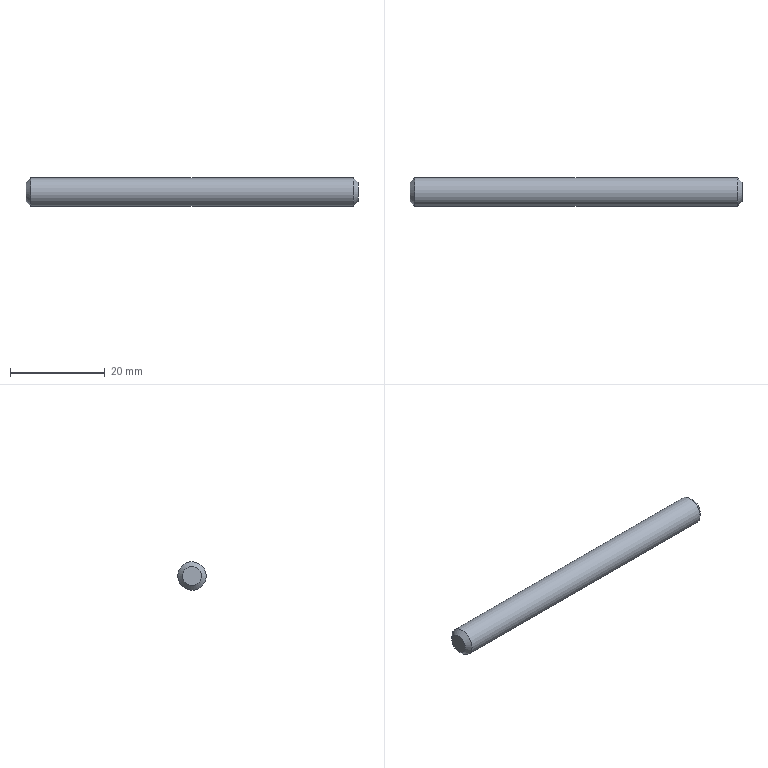Component | NX | SUPPORT | 1 solid | 5 faces | box 70 x 6 x 6 mm | volume 1962 mm3 | plane 2 | cone 2 | cylinder 1 | commonest cylinder face diameters 6 x1
STEP:
#1=CARTESIAN_POINT('',(0.,0.,0.));
#2=DIRECTION('',(0.,0.,1.));
#3=DIRECTION('',(1.,0.,0.));
#4=AXIS2_PLACEMENT_3D('',#1,#2,#3);
#5=CARTESIAN_POINT('',(-48.356,16.452,-51.303));
#6=VERTEX_POINT('',#5);
#7=CARTESIAN_POINT('',(-48.356,16.19,-48.315));
#8=DIRECTION('',(1.,0.,0.));
#9=DIRECTION('',(0.,0.08716,-0.9962));
#10=AXIS2_PLACEMENT_3D('',#7,#8,#9);
#11=CIRCLE('',#10,3.);
#12=CARTESIAN_POINT('',(20.644,16.19,-48.315));
#13=DIRECTION('',(-1.,0.,0.));
#14=DIRECTION('',(0.,-0.08716,0.9962));
#15=AXIS2_PLACEMENT_3D('',#12,#13,#14);
#16=CYLINDRICAL_SURFACE('',#15,3.);
#17=CARTESIAN_POINT('',(9.425,69.));
#18=DIRECTION('',(-1.,0.));
#19=VECTOR('',#18,1.);
#20=LINE('',#17,#19);
#21=(GEOMETRIC_REPRESENTATION_CONTEXT(2)PARAMETRIC_REPRESENTATION_CONTEXT()REPRESENTATION_CONTEXT('',''));
#22=DEFINITIONAL_REPRESENTATION('',(#20),#21);
#23=PCURVE('',#16,#22);
#24=CARTESIAN_POINT('',(-48.356,16.19,-48.315));
#25=DIRECTION('',(1.,0.,0.));
#26=DIRECTION('',(0.,0.08716,-0.9962));
#27=AXIS2_PLACEMENT_3D('',#24,#25,#26);
#28=CONICAL_SURFACE('',#27,3.,0.7854);
#29=CARTESIAN_POINT('',(0.,0.));
#30=DIRECTION('',(1.,0.));
#31=VECTOR('',#30,1.);
#32=LINE('',#29,#31);
#33=(GEOMETRIC_REPRESENTATION_CONTEXT(2)PARAMETRIC_REPRESENTATION_CONTEXT()REPRESENTATION_CONTEXT('',''));
#34=DEFINITIONAL_REPRESENTATION('',(#32),#33);
#35=PCURVE('',#28,#34);
#36=SURFACE_CURVE('',#11,(#23,#35),.PCURVE_S1.);
#37=EDGE_CURVE('',#6,#6,#36,.T.);
#38=ORIENTED_EDGE('',*,*,#37,.T.);
#39=CARTESIAN_POINT('',(19.644,16.452,-51.303));
#40=VERTEX_POINT('',#39);
#41=CARTESIAN_POINT('',(19.644,16.452,-51.303));
#42=CARTESIAN_POINT('',(-48.356,16.452,-51.303));
#43=B_SPLINE_CURVE_WITH_KNOTS('',1,(#41,#42),.UNSPECIFIED.,.F.,.F.,(2,2),(1.,69.),.PIECEWISE_BEZIER_KNOTS.);
#44=CARTESIAN_POINT('',(3.142,0.));
#45=DIRECTION('',(0.,1.));
#46=VECTOR('',#45,1.);
#47=LINE('',#44,#46);
#48=(GEOMETRIC_REPRESENTATION_CONTEXT(2)PARAMETRIC_REPRESENTATION_CONTEXT()REPRESENTATION_CONTEXT('',''));
#49=DEFINITIONAL_REPRESENTATION('',(#47),#48);
#50=PCURVE('',#16,#49);
#51=CARTESIAN_POINT('',(9.425,0.));
#52=DIRECTION('',(0.,1.));
#53=VECTOR('',#52,1.);
#54=LINE('',#51,#53);
#55=(GEOMETRIC_REPRESENTATION_CONTEXT(2)PARAMETRIC_REPRESENTATION_CONTEXT()REPRESENTATION_CONTEXT('',''));
#56=DEFINITIONAL_REPRESENTATION('',(#54),#55);
#57=PCURVE('',#16,#56);
#58=SEAM_CURVE('',#43,(#50,#57),.PCURVE_S1.);
#59=EDGE_CURVE('',#40,#6,#58,.T.);
#60=ORIENTED_EDGE('',*,*,#59,.F.);
#61=CARTESIAN_POINT('',(19.644,16.19,-48.315));
#62=DIRECTION('',(-1.,0.,0.));
#63=DIRECTION('',(0.,0.08716,-0.9962));
#64=AXIS2_PLACEMENT_3D('',#61,#62,#63);
#65=CIRCLE('',#64,3.);
#66=CARTESIAN_POINT('',(3.142,1.));
#67=DIRECTION('',(1.,0.));
#68=VECTOR('',#67,1.);
#69=LINE('',#66,#68);
#70=(GEOMETRIC_REPRESENTATION_CONTEXT(2)PARAMETRIC_REPRESENTATION_CONTEXT()REPRESENTATION_CONTEXT('',''));
#71=DEFINITIONAL_REPRESENTATION('',(#69),#70);
#72=PCURVE('',#16,#71);
#73=CARTESIAN_POINT('',(20.644,16.19,-48.315));
#74=DIRECTION('',(-1.,0.,0.));
#75=DIRECTION('',(0.,-0.08716,0.9962));
#76=AXIS2_PLACEMENT_3D('',#73,#74,#75);
#77=CONICAL_SURFACE('',#76,2.,0.7854);
#78=CARTESIAN_POINT('',(3.142,1.));
#79=DIRECTION('',(1.,0.));
#80=VECTOR('',#79,1.);
#81=LINE('',#78,#80);
#82=(GEOMETRIC_REPRESENTATION_CONTEXT(2)PARAMETRIC_REPRESENTATION_CONTEXT()REPRESENTATION_CONTEXT('',''));
#83=DEFINITIONAL_REPRESENTATION('',(#81),#82);
#84=PCURVE('',#77,#83);
#85=SURFACE_CURVE('',#65,(#72,#84),.PCURVE_S1.);
#86=EDGE_CURVE('',#40,#40,#85,.T.);
#87=ORIENTED_EDGE('',*,*,#86,.T.);
#88=ORIENTED_EDGE('',*,*,#59,.T.);
#89=EDGE_LOOP('',(#38,#60,#87,#88));
#90=FACE_BOUND('',#89,.T.);
#91=ADVANCED_FACE('',(#90),#16,.T.);
#92=CARTESIAN_POINT('',(20.644,16.365,-50.307));
#93=VERTEX_POINT('',#92);
#94=CARTESIAN_POINT('',(20.644,16.19,-48.315));
#95=DIRECTION('',(1.,0.,0.));
#96=DIRECTION('',(0.,0.08716,-0.9962));
#97=AXIS2_PLACEMENT_3D('',#94,#95,#96);
#98=CIRCLE('',#97,2.);
#99=CARTESIAN_POINT('',(20.644,16.19,-48.315));
#100=DIRECTION('',(1.,0.,0.));
#101=DIRECTION('',(0.,0.08716,-0.9962));
#102=AXIS2_PLACEMENT_3D('',#99,#100,#101);
#103=PLANE('',#102);
#104=CARTESIAN_POINT('',(0.,0.));
#105=DIRECTION('',(1.,0.));
#106=AXIS2_PLACEMENT_2D('',#104,#105);
#107=CIRCLE('',#106,2.);
#108=(GEOMETRIC_REPRESENTATION_CONTEXT(2)PARAMETRIC_REPRESENTATION_CONTEXT()REPRESENTATION_CONTEXT('',''));
#109=DEFINITIONAL_REPRESENTATION('',(#107),#108);
#110=PCURVE('',#103,#109);
#111=CARTESIAN_POINT('',(9.425,0.));
#112=DIRECTION('',(-1.,0.));
#113=VECTOR('',#112,1.);
#114=LINE('',#111,#113);
#115=(GEOMETRIC_REPRESENTATION_CONTEXT(2)PARAMETRIC_REPRESENTATION_CONTEXT()REPRESENTATION_CONTEXT('',''));
#116=DEFINITIONAL_REPRESENTATION('',(#114),#115);
#117=PCURVE('',#77,#116);
#118=SURFACE_CURVE('',#98,(#110,#117),.PCURVE_S1.);
#119=EDGE_CURVE('',#93,#93,#118,.T.);
#120=ORIENTED_EDGE('',*,*,#119,.T.);
#121=EDGE_LOOP('',(#120));
#122=FACE_BOUND('',#121,.T.);
#123=ADVANCED_FACE('',(#122),#103,.T.);
#124=CARTESIAN_POINT('',(-49.356,16.365,-50.307));
#125=VERTEX_POINT('',#124);
#126=CARTESIAN_POINT('',(-49.356,16.19,-48.315));
#127=DIRECTION('',(-1.,0.,0.));
#128=DIRECTION('',(0.,0.08716,-0.9962));
#129=AXIS2_PLACEMENT_3D('',#126,#127,#128);
#130=CIRCLE('',#129,2.);
#131=CARTESIAN_POINT('',(-49.356,16.19,-48.315));
#132=DIRECTION('',(1.,0.,0.));
#133=DIRECTION('',(0.,0.08716,-0.9962));
#134=AXIS2_PLACEMENT_3D('',#131,#132,#133);
#135=PLANE('',#134);
#136=CARTESIAN_POINT('',(2.,0.));
#137=CARTESIAN_POINT('',(2.,-3.464));
#138=CARTESIAN_POINT('',(-1.,-1.732));
#139=CARTESIAN_POINT('',(-4.,-0.));
#140=CARTESIAN_POINT('',(-1.,1.732));
#141=CARTESIAN_POINT('',(2.,3.464));
#142=CARTESIAN_POINT('',(2.,0.));
#143=(BOUNDED_CURVE()B_SPLINE_CURVE(2,(#136,#137,#138,#139,#140,#141,#142),.UNSPECIFIED.,.T.,.F.)B_SPLINE_CURVE_WITH_KNOTS((1,2,2,2,2,1),(-2.094,0.,2.094,4.189,6.283,8.378),.UNSPECIFIED.)CURVE()GEOMETRIC_REPRESENTATION_ITEM()RATIONAL_B_SPLINE_CURVE((1.,0.5,1.,0.5,1.,0.5,1.))REPRESENTATION_ITEM(''));
#144=(GEOMETRIC_REPRESENTATION_CONTEXT(2)PARAMETRIC_REPRESENTATION_CONTEXT()REPRESENTATION_CONTEXT('',''));
#145=DEFINITIONAL_REPRESENTATION('',(#143),#144);
#146=PCURVE('',#135,#145);
#147=CARTESIAN_POINT('',(6.283,-1.));
#148=DIRECTION('',(-1.,0.));
#149=VECTOR('',#148,1.);
#150=LINE('',#147,#149);
#151=(GEOMETRIC_REPRESENTATION_CONTEXT(2)PARAMETRIC_REPRESENTATION_CONTEXT()REPRESENTATION_CONTEXT('',''));
#152=DEFINITIONAL_REPRESENTATION('',(#150),#151);
#153=PCURVE('',#28,#152);
#154=SURFACE_CURVE('',#130,(#146,#153),.PCURVE_S1.);
#155=EDGE_CURVE('',#125,#125,#154,.T.);
#156=ORIENTED_EDGE('',*,*,#155,.T.);
#157=EDGE_LOOP('',(#156));
#158=FACE_BOUND('',#157,.T.);
#159=ADVANCED_FACE('',(#158),#135,.F.);
#160=ORIENTED_EDGE('',*,*,#155,.F.);
#161=CARTESIAN_POINT('',(-49.356,16.365,-50.307));
#162=CARTESIAN_POINT('',(-48.356,16.452,-51.303));
#163=B_SPLINE_CURVE_WITH_KNOTS('',1,(#161,#162),.UNSPECIFIED.,.F.,.F.,(2,2),(-1.414,0.),.PIECEWISE_BEZIER_KNOTS.);
#164=CARTESIAN_POINT('',(6.283,0.));
#165=DIRECTION('',(0.,1.));
#166=VECTOR('',#165,1.);
#167=LINE('',#164,#166);
#168=(GEOMETRIC_REPRESENTATION_CONTEXT(2)PARAMETRIC_REPRESENTATION_CONTEXT()REPRESENTATION_CONTEXT('',''));
#169=DEFINITIONAL_REPRESENTATION('',(#167),#168);
#170=PCURVE('',#28,#169);
#171=CARTESIAN_POINT('',(0.,0.));
#172=DIRECTION('',(0.,1.));
#173=VECTOR('',#172,1.);
#174=LINE('',#171,#173);
#175=(GEOMETRIC_REPRESENTATION_CONTEXT(2)PARAMETRIC_REPRESENTATION_CONTEXT()REPRESENTATION_CONTEXT('',''));
#176=DEFINITIONAL_REPRESENTATION('',(#174),#175);
#177=PCURVE('',#28,#176);
#178=SEAM_CURVE('',#163,(#170,#177),.PCURVE_S1.);
#179=EDGE_CURVE('',#125,#6,#178,.T.);
#180=ORIENTED_EDGE('',*,*,#179,.T.);
#181=ORIENTED_EDGE('',*,*,#37,.F.);
#182=ORIENTED_EDGE('',*,*,#179,.F.);
#183=EDGE_LOOP('',(#160,#180,#181,#182));
#184=FACE_BOUND('',#183,.T.);
#185=ADVANCED_FACE('',(#184),#28,.T.);
#186=ORIENTED_EDGE('',*,*,#86,.F.);
#187=CARTESIAN_POINT('',(20.644,16.365,-50.307));
#188=CARTESIAN_POINT('',(19.644,16.452,-51.303));
#189=B_SPLINE_CURVE_WITH_KNOTS('',1,(#187,#188),.UNSPECIFIED.,.F.,.F.,(2,2),(0.,1.414),.PIECEWISE_BEZIER_KNOTS.);
#190=CARTESIAN_POINT('',(3.142,0.));
#191=DIRECTION('',(0.,1.));
#192=VECTOR('',#191,1.);
#193=LINE('',#190,#192);
#194=(GEOMETRIC_REPRESENTATION_CONTEXT(2)PARAMETRIC_REPRESENTATION_CONTEXT()REPRESENTATION_CONTEXT('',''));
#195=DEFINITIONAL_REPRESENTATION('',(#193),#194);
#196=PCURVE('',#77,#195);
#197=CARTESIAN_POINT('',(9.425,0.));
#198=DIRECTION('',(0.,1.));
#199=VECTOR('',#198,1.);
#200=LINE('',#197,#199);
#201=(GEOMETRIC_REPRESENTATION_CONTEXT(2)PARAMETRIC_REPRESENTATION_CONTEXT()REPRESENTATION_CONTEXT('',''));
#202=DEFINITIONAL_REPRESENTATION('',(#200),#201);
#203=PCURVE('',#77,#202);
#204=SEAM_CURVE('',#189,(#196,#203),.PCURVE_S1.);
#205=EDGE_CURVE('',#93,#40,#204,.T.);
#206=ORIENTED_EDGE('',*,*,#205,.F.);
#207=ORIENTED_EDGE('',*,*,#119,.F.);
#208=ORIENTED_EDGE('',*,*,#205,.T.);
#209=EDGE_LOOP('',(#186,#206,#207,#208));
#210=FACE_BOUND('',#209,.T.);
#211=ADVANCED_FACE('',(#210),#77,.T.);
#212=CLOSED_SHELL('',(#91,#123,#159,#185,#211));
#213=MANIFOLD_SOLID_BREP('',#212);
#214=(LENGTH_UNIT()NAMED_UNIT(*)SI_UNIT(.MILLI.,.METRE.));
#215=UNCERTAINTY_MEASURE_WITH_UNIT(LENGTH_MEASURE(0.00001),#214,'','');
#216=(NAMED_UNIT(*)PLANE_ANGLE_UNIT()SI_UNIT($,.RADIAN.));
#217=(NAMED_UNIT(*)SI_UNIT($,.STERADIAN.)SOLID_ANGLE_UNIT());
#218=(GEOMETRIC_REPRESENTATION_CONTEXT(3)GLOBAL_UNCERTAINTY_ASSIGNED_CONTEXT((#215))GLOBAL_UNIT_ASSIGNED_CONTEXT((#214,#216,#217))REPRESENTATION_CONTEXT('',''));
#219=ADVANCED_BREP_SHAPE_REPRESENTATION('',(#4,#213),#218);